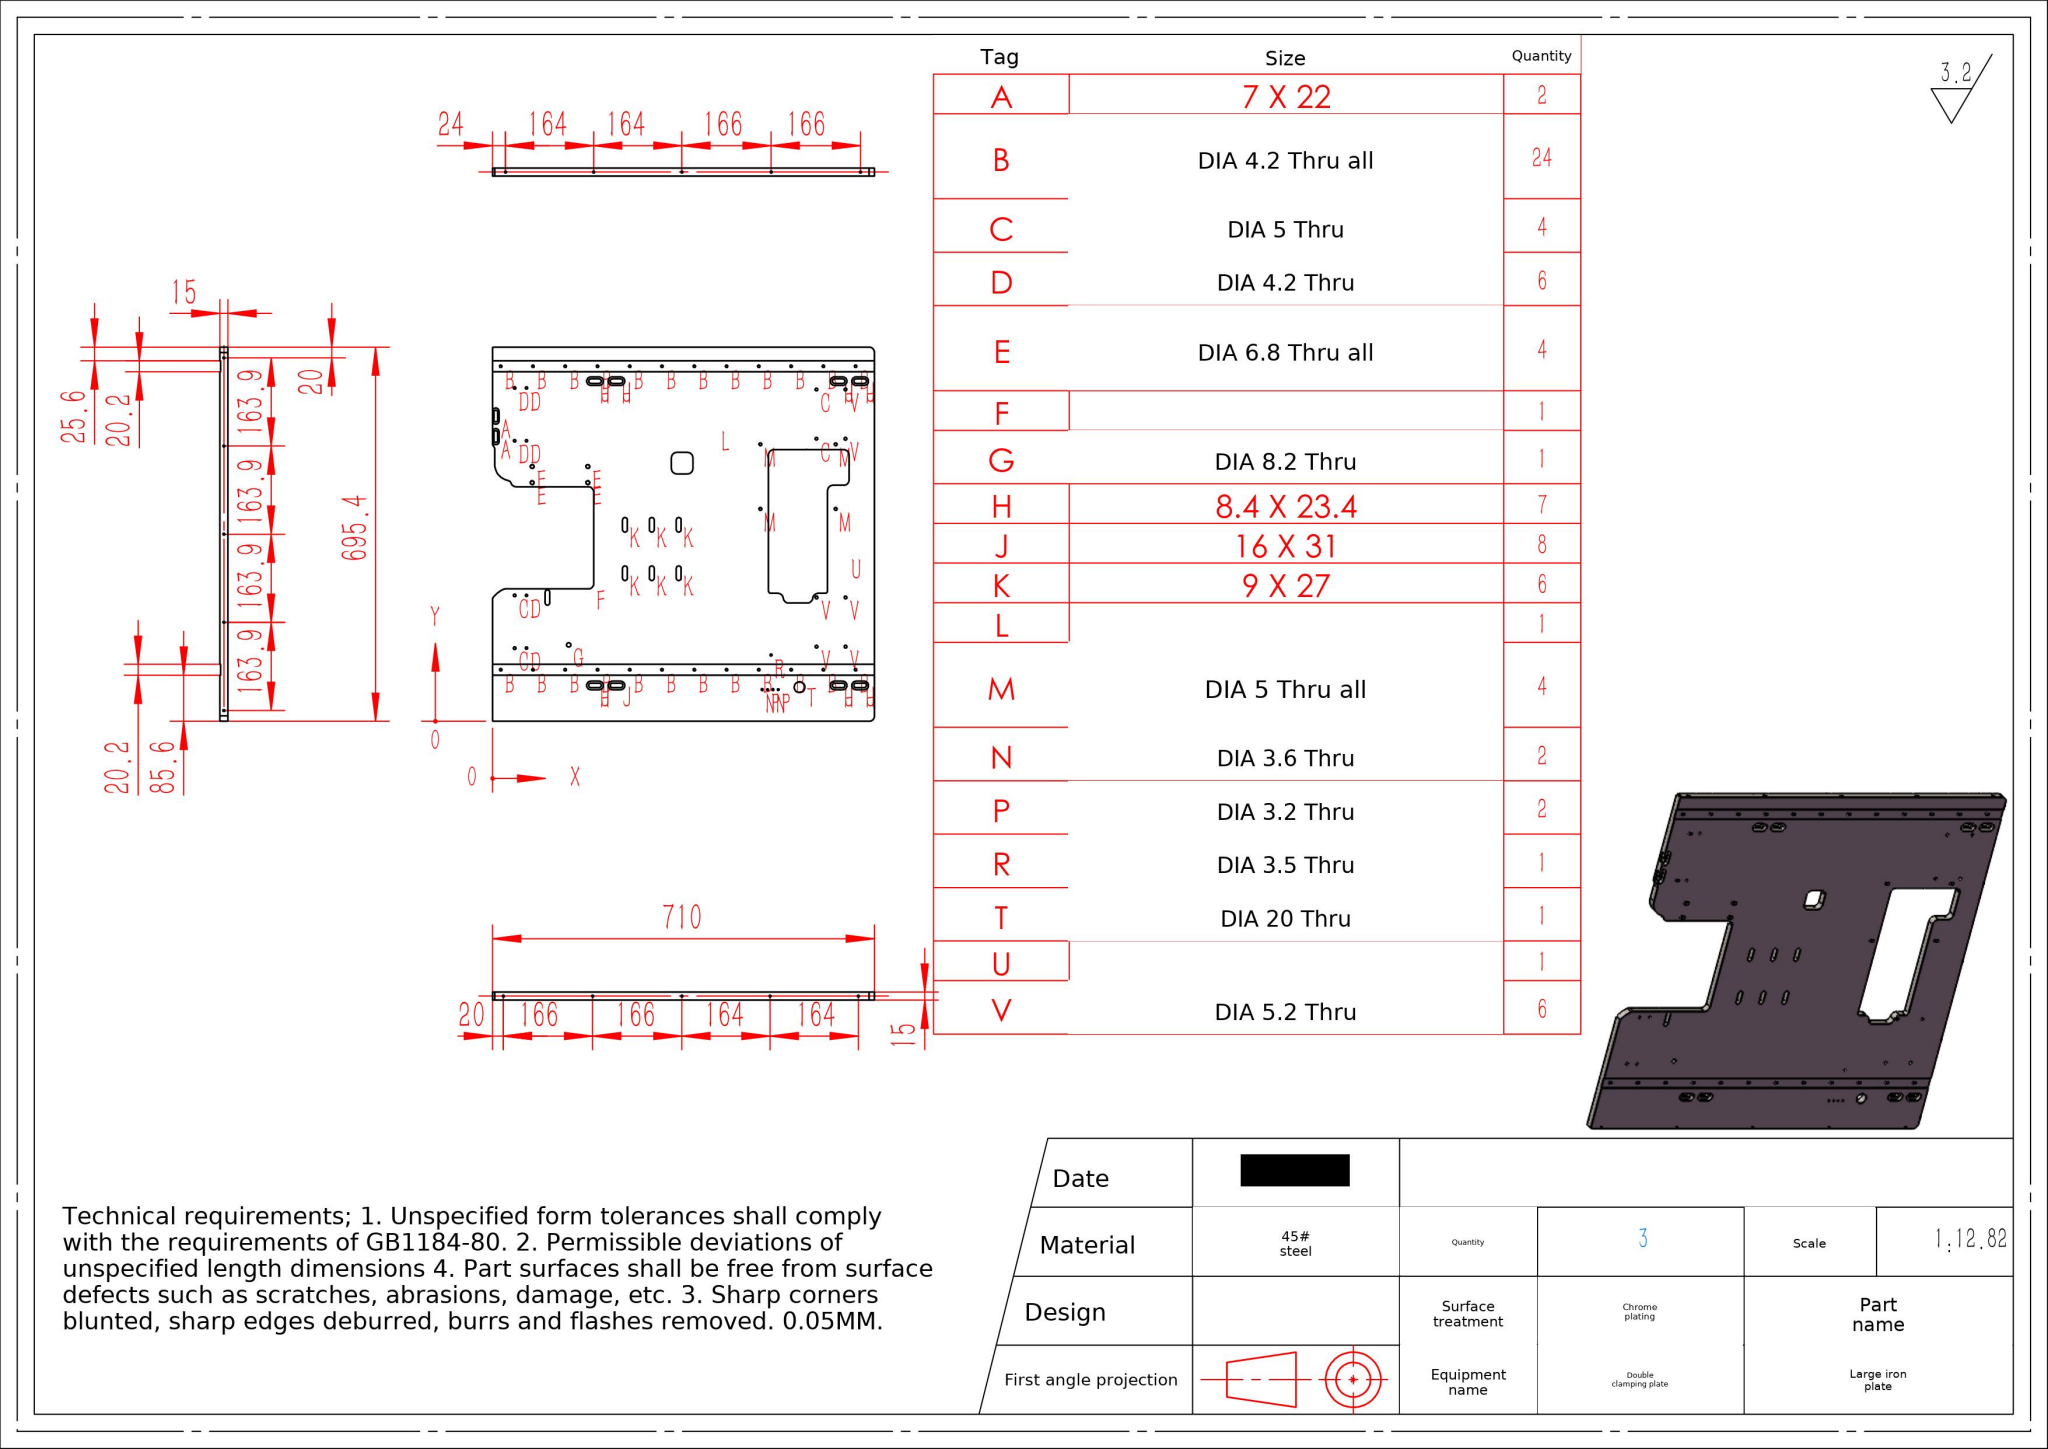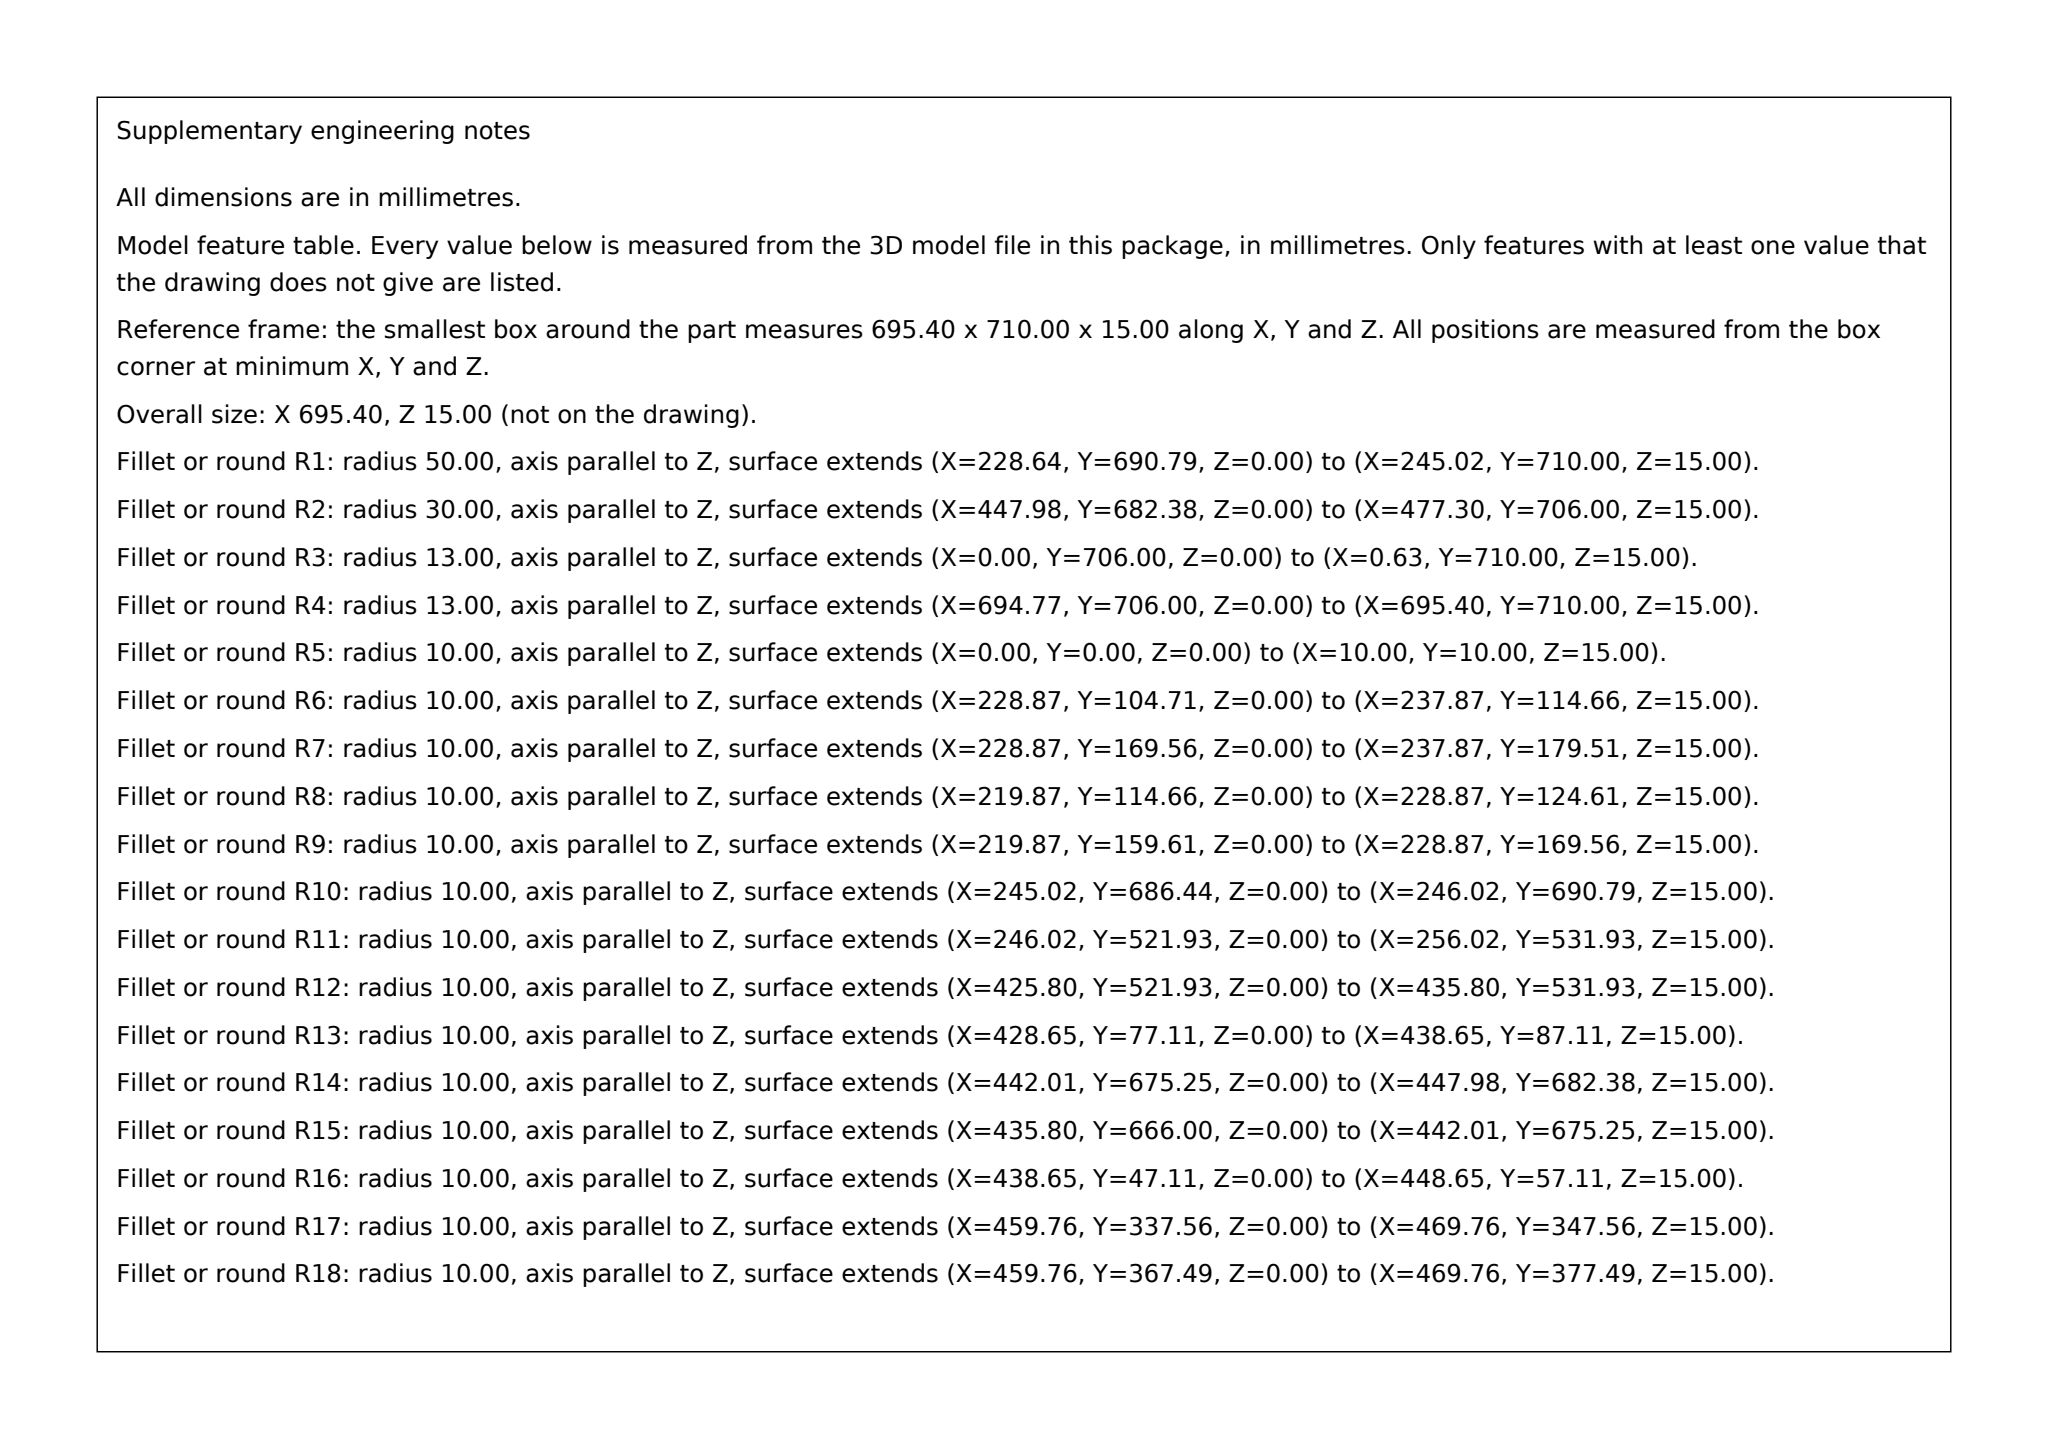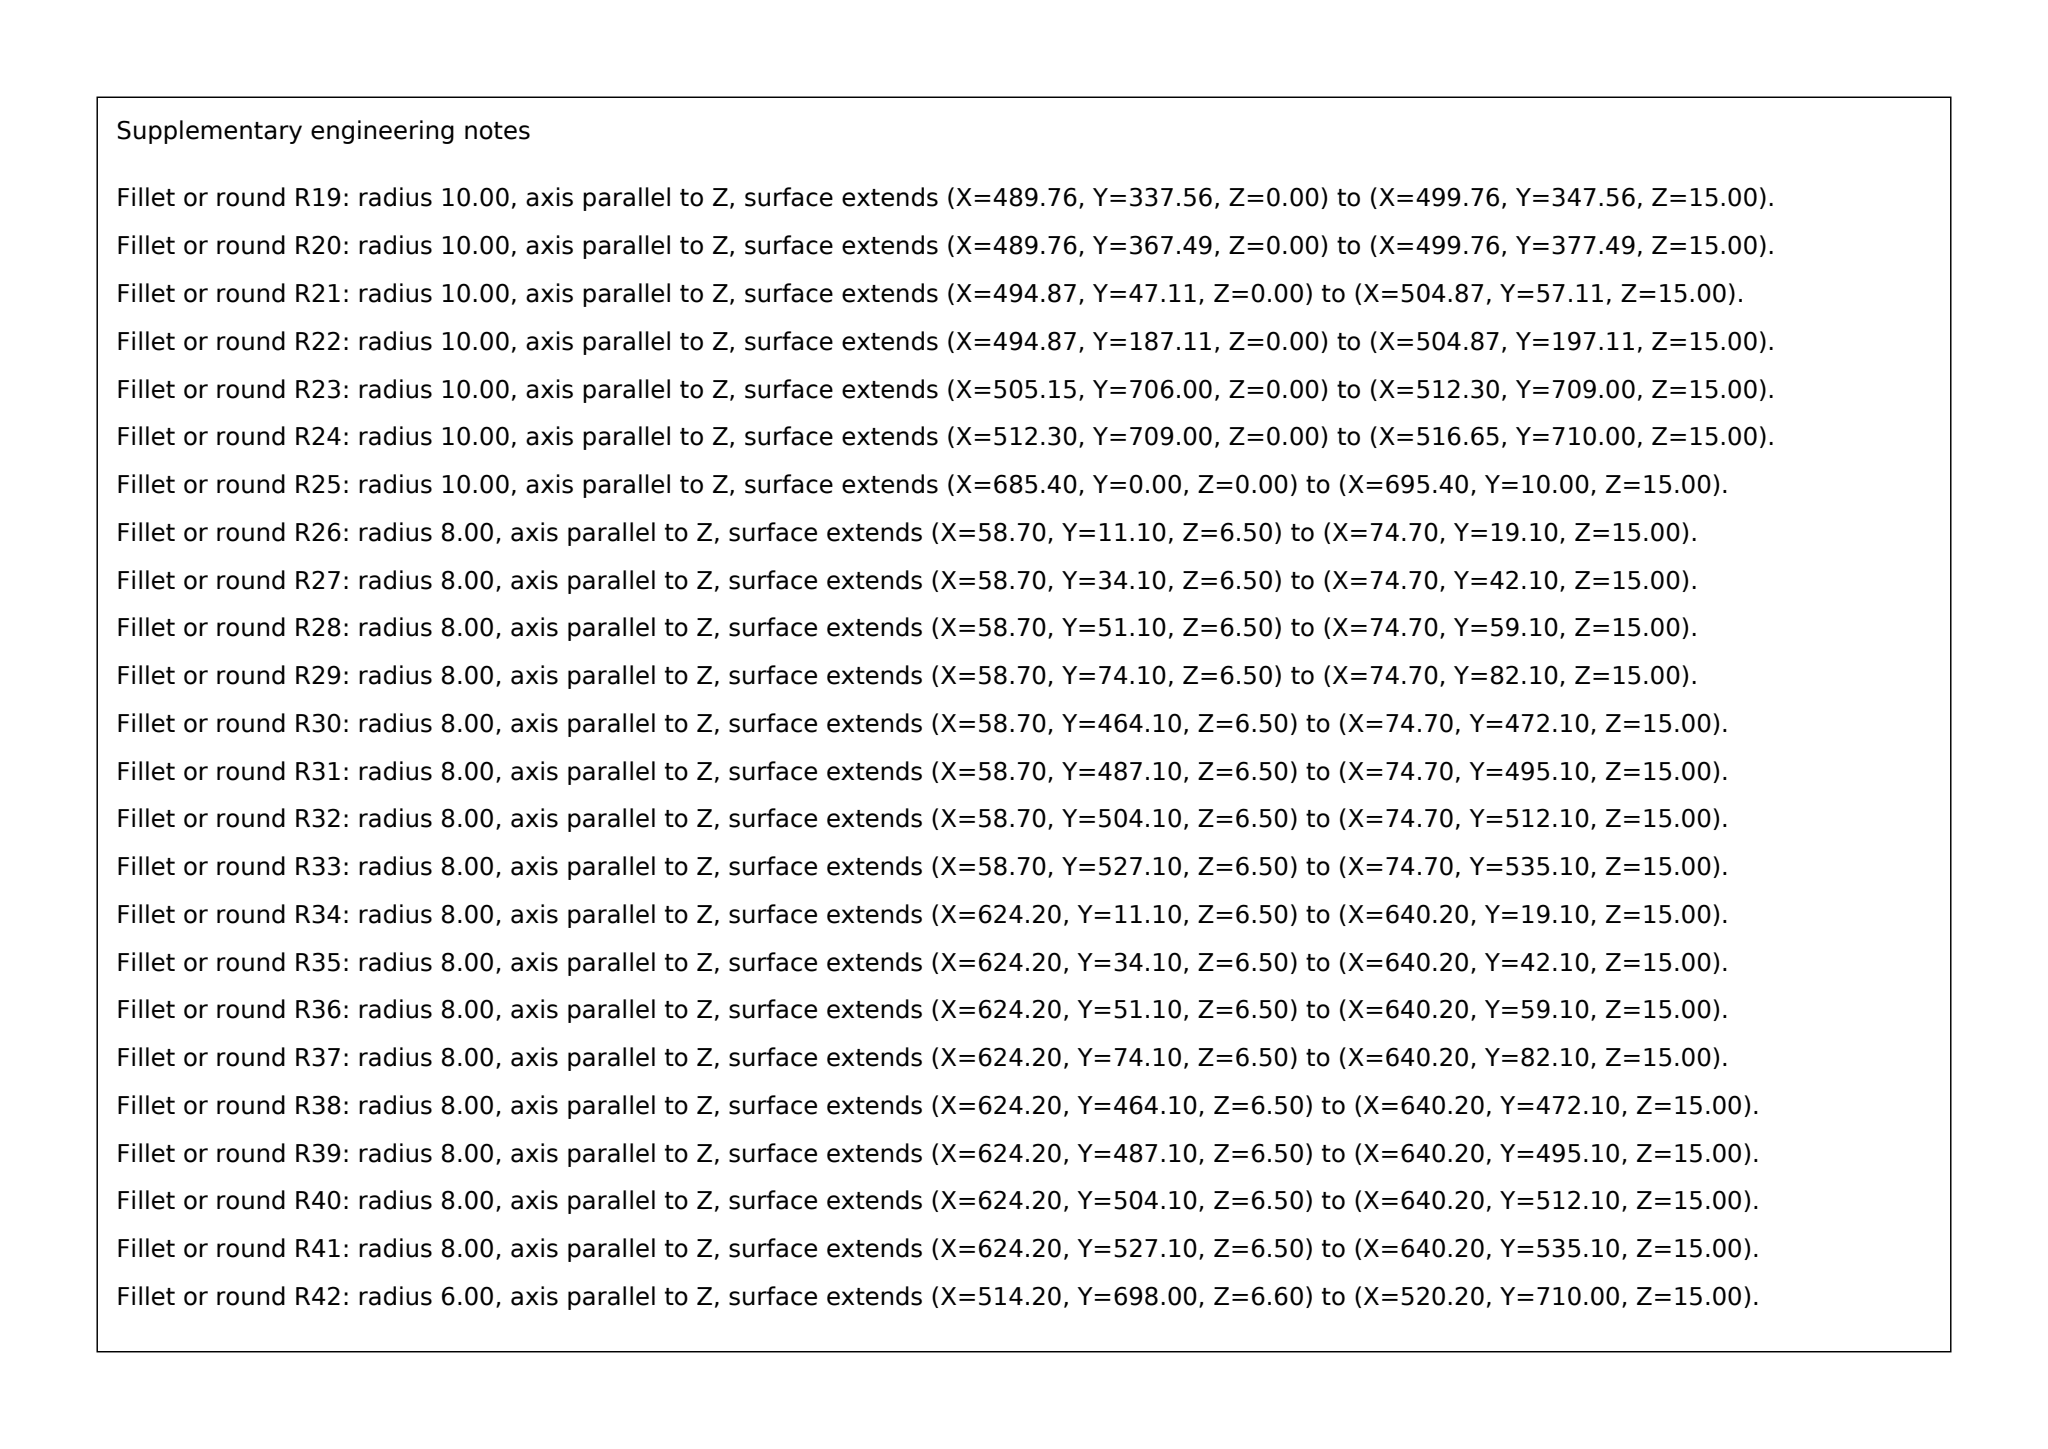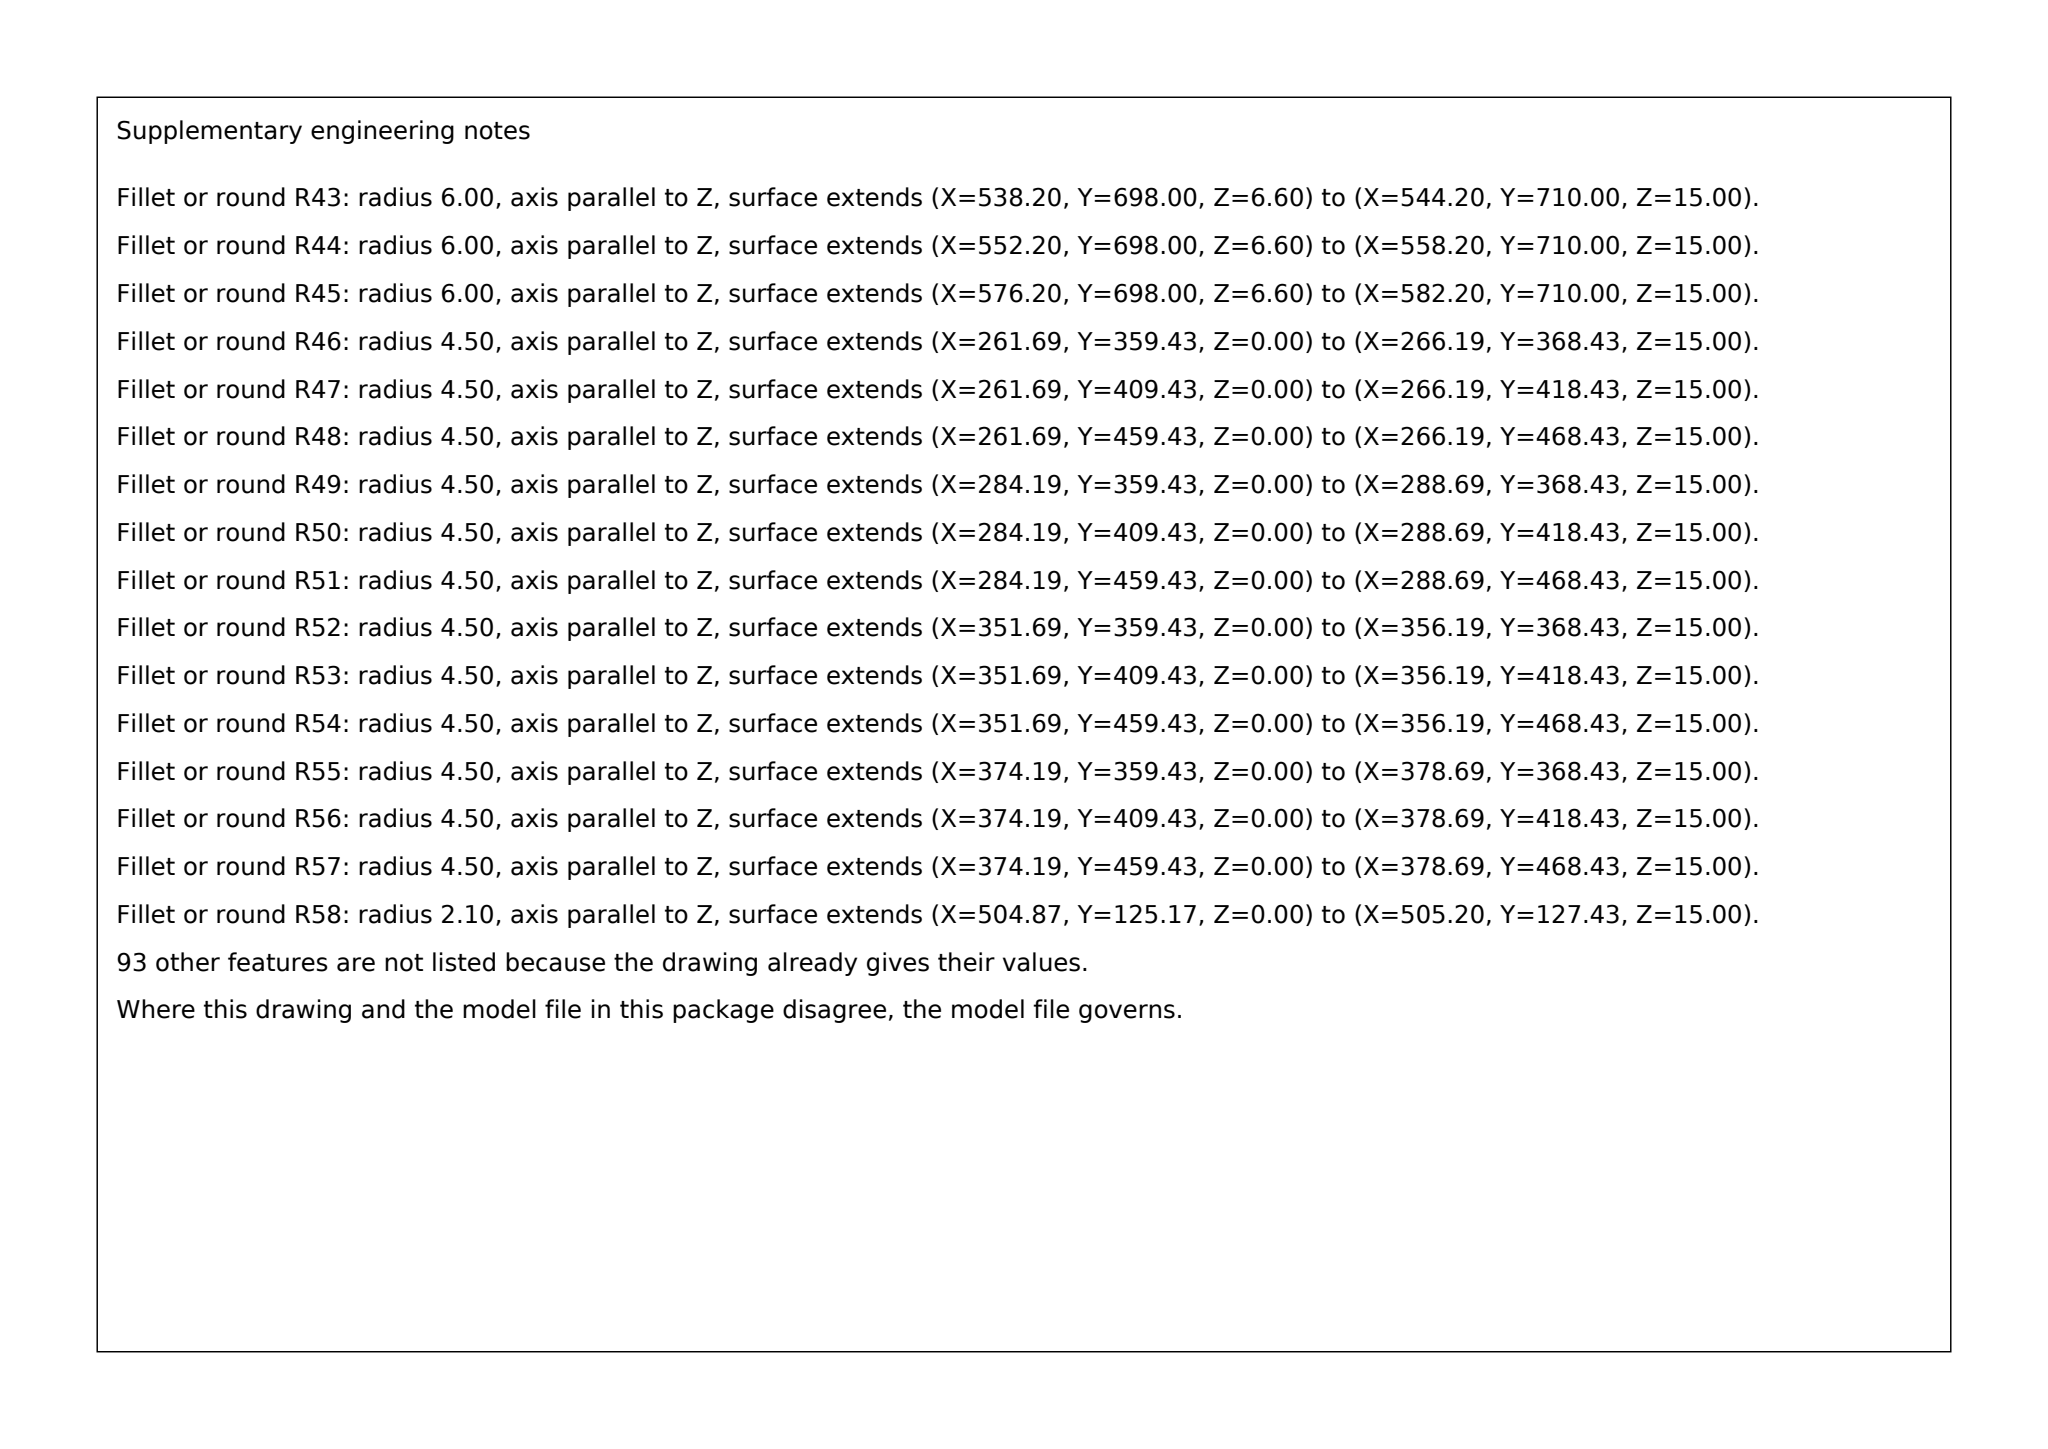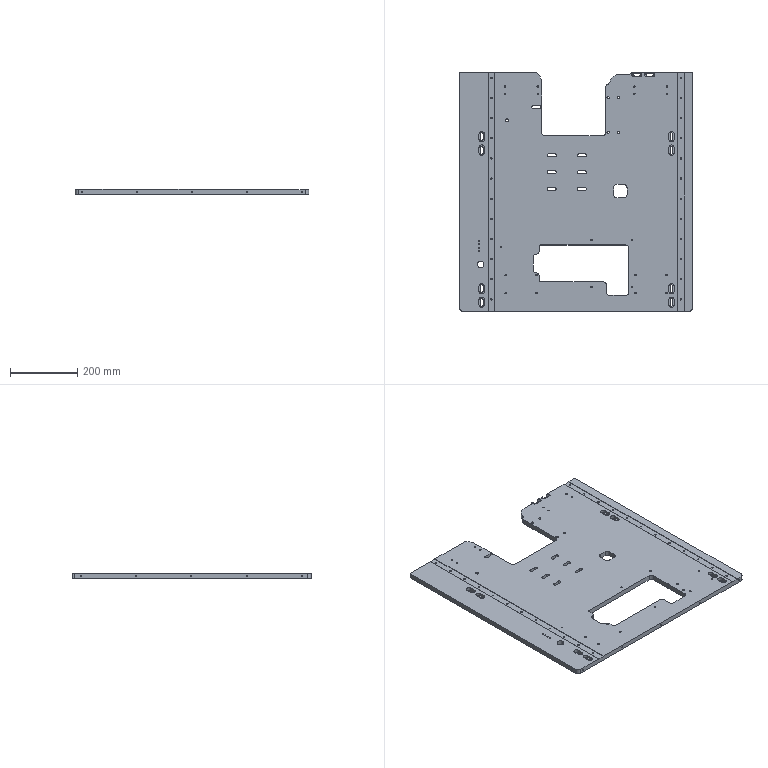Part | SolidWorks | mm | material 45# steel | 1 solid | 357 faces | box 695.4 x 710 x 15 mm | volume 6205268 mm3 | cylinder 233 | plane 94 | cone 30 | commonest cylinder face diameters 4.2 x61 3.3 x30 20 x23 9 x18 5 x16 8.4 x16 16 x16 5.2 x12